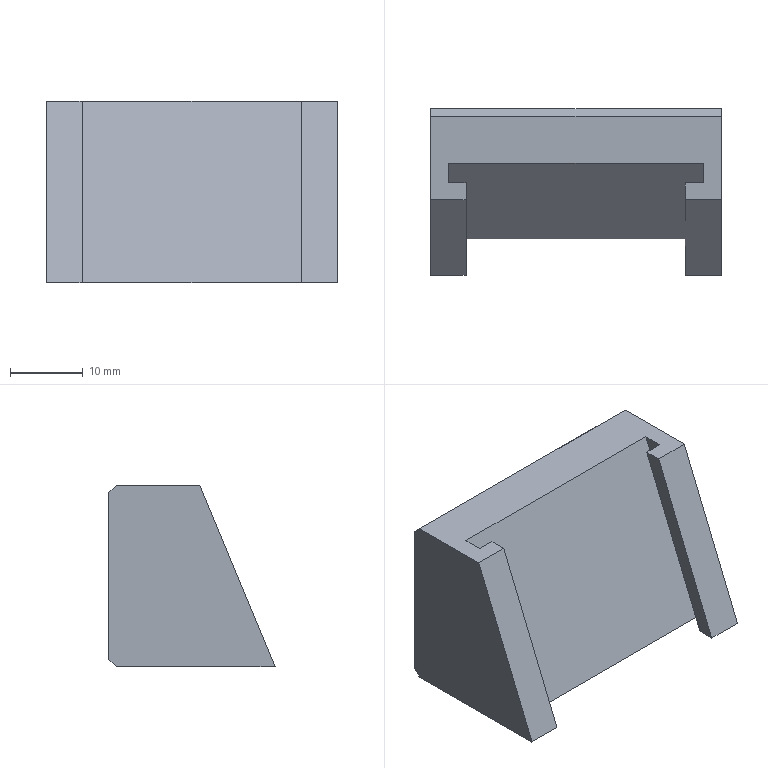Component | NX | CLAMP_SLIDER | 1 solid | 16 faces | box 40 x 22.86 x 25 mm | volume 13543 mm3 | plane 16
STEP:
#1=CARTESIAN_POINT('',(0.,0.,0.));
#2=DIRECTION('',(0.,0.,1.));
#3=DIRECTION('',(1.,0.,0.));
#4=AXIS2_PLACEMENT_3D('',#1,#2,#3);
#5=CARTESIAN_POINT('',(146.772,200.315,195.246));
#6=VERTEX_POINT('',#5);
#7=CARTESIAN_POINT('',(141.898,200.315,195.246));
#8=VERTEX_POINT('',#7);
#9=CARTESIAN_POINT('',(181.898,200.315,195.246));
#10=DIRECTION('',(-1.,0.,0.));
#11=VECTOR('',#10,1.);
#12=LINE('',#9,#11);
#13=CARTESIAN_POINT('',(181.898,200.315,195.246));
#14=DIRECTION('',(0.,-0.9239,0.3827));
#15=DIRECTION('',(0.,0.3827,0.9239));
#16=AXIS2_PLACEMENT_3D('',#13,#14,#15);
#17=PLANE('',#16);
#18=CARTESIAN_POINT('',(0.,0.));
#19=DIRECTION('',(0.,1.));
#20=VECTOR('',#19,1.);
#21=LINE('',#18,#20);
#22=(GEOMETRIC_REPRESENTATION_CONTEXT(2)PARAMETRIC_REPRESENTATION_CONTEXT()REPRESENTATION_CONTEXT('',''));
#23=DEFINITIONAL_REPRESENTATION('',(#21),#22);
#24=PCURVE('',#17,#23);
#25=CARTESIAN_POINT('',(181.898,222.171,195.246));
#26=DIRECTION('',(0.,0.,-1.));
#27=DIRECTION('',(1.,0.,0.));
#28=AXIS2_PLACEMENT_3D('',#25,#26,#27);
#29=PLANE('',#28);
#30=CARTESIAN_POINT('',(0.,21.855));
#31=DIRECTION('',(-1.,0.));
#32=VECTOR('',#31,1.);
#33=LINE('',#30,#32);
#34=(GEOMETRIC_REPRESENTATION_CONTEXT(2)PARAMETRIC_REPRESENTATION_CONTEXT()REPRESENTATION_CONTEXT('',''));
#35=DEFINITIONAL_REPRESENTATION('',(#33),#34);
#36=PCURVE('',#29,#35);
#37=SURFACE_CURVE('',#12,(#24,#36),.PCURVE_S1.);
#38=EDGE_CURVE('',#6,#8,#37,.T.);
#39=ORIENTED_EDGE('',*,*,#38,.F.);
#40=CARTESIAN_POINT('',(146.772,210.671,220.246));
#41=VERTEX_POINT('',#40);
#42=CARTESIAN_POINT('',(146.772,195.363,183.291));
#43=DIRECTION('',(0.,0.3827,0.9239));
#44=VECTOR('',#43,1.);
#45=LINE('',#42,#44);
#46=CARTESIAN_POINT('',(-12.94,35.126));
#47=DIRECTION('',(1.,0.));
#48=VECTOR('',#47,1.);
#49=LINE('',#46,#48);
#50=(GEOMETRIC_REPRESENTATION_CONTEXT(2)PARAMETRIC_REPRESENTATION_CONTEXT()REPRESENTATION_CONTEXT('',''));
#51=DEFINITIONAL_REPRESENTATION('',(#49),#50);
#52=PCURVE('',#17,#51);
#53=CARTESIAN_POINT('',(146.772,197.663,183.291));
#54=DIRECTION('',(-1.,-0.00001531,0.00000634));
#55=DIRECTION('',(0.00001531,-1.,-0.));
#56=AXIS2_PLACEMENT_3D('',#53,#54,#55);
#57=PLANE('',#56);
#58=CARTESIAN_POINT('',(2.3,0.));
#59=DIRECTION('',(-0.3827,0.9239));
#60=VECTOR('',#59,1.);
#61=LINE('',#58,#60);
#62=(GEOMETRIC_REPRESENTATION_CONTEXT(2)PARAMETRIC_REPRESENTATION_CONTEXT()REPRESENTATION_CONTEXT('',''));
#63=DEFINITIONAL_REPRESENTATION('',(#61),#62);
#64=PCURVE('',#57,#63);
#65=SURFACE_CURVE('',#45,(#52,#64),.PCURVE_S1.);
#66=EDGE_CURVE('',#6,#41,#65,.T.);
#67=ORIENTED_EDGE('',*,*,#66,.T.);
#68=CARTESIAN_POINT('',(141.898,210.671,220.246));
#69=VERTEX_POINT('',#68);
#70=CARTESIAN_POINT('',(181.898,210.671,220.246));
#71=DIRECTION('',(-1.,0.,0.));
#72=VECTOR('',#71,1.);
#73=LINE('',#70,#72);
#74=CARTESIAN_POINT('',(27.06,0.));
#75=DIRECTION('',(0.,1.));
#76=VECTOR('',#75,1.);
#77=LINE('',#74,#76);
#78=(GEOMETRIC_REPRESENTATION_CONTEXT(2)PARAMETRIC_REPRESENTATION_CONTEXT()REPRESENTATION_CONTEXT('',''));
#79=DEFINITIONAL_REPRESENTATION('',(#77),#78);
#80=PCURVE('',#17,#79);
#81=CARTESIAN_POINT('',(181.898,210.671,220.246));
#82=DIRECTION('',(0.,0.,1.));
#83=DIRECTION('',(-1.,0.,0.));
#84=AXIS2_PLACEMENT_3D('',#81,#82,#83);
#85=PLANE('',#84);
#86=CARTESIAN_POINT('',(0.,0.));
#87=DIRECTION('',(1.,0.));
#88=VECTOR('',#87,1.);
#89=LINE('',#86,#88);
#90=(GEOMETRIC_REPRESENTATION_CONTEXT(2)PARAMETRIC_REPRESENTATION_CONTEXT()REPRESENTATION_CONTEXT('',''));
#91=DEFINITIONAL_REPRESENTATION('',(#89),#90);
#92=PCURVE('',#85,#91);
#93=SURFACE_CURVE('',#73,(#80,#92),.PCURVE_S1.);
#94=EDGE_CURVE('',#41,#69,#93,.T.);
#95=ORIENTED_EDGE('',*,*,#94,.T.);
#96=CARTESIAN_POINT('',(141.898,200.315,195.246));
#97=DIRECTION('',(0.,0.3827,0.9239));
#98=VECTOR('',#97,1.);
#99=LINE('',#96,#98);
#100=CARTESIAN_POINT('',(0.,40.));
#101=DIRECTION('',(1.,0.));
#102=VECTOR('',#101,1.);
#103=LINE('',#100,#102);
#104=(GEOMETRIC_REPRESENTATION_CONTEXT(2)PARAMETRIC_REPRESENTATION_CONTEXT()REPRESENTATION_CONTEXT('',''));
#105=DEFINITIONAL_REPRESENTATION('',(#103),#104);
#106=PCURVE('',#17,#105);
#107=CARTESIAN_POINT('',(141.898,223.171,220.246));
#108=DIRECTION('',(-1.,0.,0.));
#109=DIRECTION('',(0.,0.,-1.));
#110=AXIS2_PLACEMENT_3D('',#107,#108,#109);
#111=PLANE('',#110);
#112=CARTESIAN_POINT('',(25.,22.855));
#113=DIRECTION('',(-0.9239,-0.3827));
#114=VECTOR('',#113,1.);
#115=LINE('',#112,#114);
#116=(GEOMETRIC_REPRESENTATION_CONTEXT(2)PARAMETRIC_REPRESENTATION_CONTEXT()REPRESENTATION_CONTEXT('',''));
#117=DEFINITIONAL_REPRESENTATION('',(#115),#116);
#118=PCURVE('',#111,#117);
#119=SURFACE_CURVE('',#99,(#106,#118),.PCURVE_S1.);
#120=EDGE_CURVE('',#8,#69,#119,.T.);
#121=ORIENTED_EDGE('',*,*,#120,.F.);
#122=EDGE_LOOP('',(#39,#67,#95,#121));
#123=FACE_BOUND('',#122,.T.);
#124=ADVANCED_FACE('',(#123),#17,.T.);
#125=CARTESIAN_POINT('',(141.898,223.171,219.246));
#126=VERTEX_POINT('',#125);
#127=CARTESIAN_POINT('',(141.898,223.171,196.246));
#128=VERTEX_POINT('',#127);
#129=CARTESIAN_POINT('',(141.898,223.171,219.246));
#130=DIRECTION('',(0.,0.,-1.));
#131=VECTOR('',#130,1.);
#132=LINE('',#129,#131);
#133=CARTESIAN_POINT('',(181.898,223.171,219.246));
#134=DIRECTION('',(0.,1.,0.));
#135=DIRECTION('',(0.,0.,-1.));
#136=AXIS2_PLACEMENT_3D('',#133,#134,#135);
#137=PLANE('',#136);
#138=CARTESIAN_POINT('',(0.,40.));
#139=DIRECTION('',(1.,0.));
#140=VECTOR('',#139,1.);
#141=LINE('',#138,#140);
#142=(GEOMETRIC_REPRESENTATION_CONTEXT(2)PARAMETRIC_REPRESENTATION_CONTEXT()REPRESENTATION_CONTEXT('',''));
#143=DEFINITIONAL_REPRESENTATION('',(#141),#142);
#144=PCURVE('',#137,#143);
#145=CARTESIAN_POINT('',(1.,0.));
#146=DIRECTION('',(1.,-0.));
#147=VECTOR('',#146,1.);
#148=LINE('',#145,#147);
#149=(GEOMETRIC_REPRESENTATION_CONTEXT(2)PARAMETRIC_REPRESENTATION_CONTEXT()REPRESENTATION_CONTEXT('',''));
#150=DEFINITIONAL_REPRESENTATION('',(#148),#149);
#151=PCURVE('',#111,#150);
#152=SURFACE_CURVE('',#132,(#144,#151),.PCURVE_S1.);
#153=EDGE_CURVE('',#126,#128,#152,.T.);
#154=ORIENTED_EDGE('',*,*,#153,.F.);
#155=CARTESIAN_POINT('',(181.898,223.171,219.246));
#156=VERTEX_POINT('',#155);
#157=CARTESIAN_POINT('',(181.898,223.171,219.246));
#158=DIRECTION('',(-1.,0.,0.));
#159=VECTOR('',#158,1.);
#160=LINE('',#157,#159);
#161=CARTESIAN_POINT('',(0.,0.));
#162=DIRECTION('',(0.,1.));
#163=VECTOR('',#162,1.);
#164=LINE('',#161,#163);
#165=(GEOMETRIC_REPRESENTATION_CONTEXT(2)PARAMETRIC_REPRESENTATION_CONTEXT()REPRESENTATION_CONTEXT('',''));
#166=DEFINITIONAL_REPRESENTATION('',(#164),#165);
#167=PCURVE('',#137,#166);
#168=CARTESIAN_POINT('',(181.898,222.171,220.246));
#169=DIRECTION('',(0.,0.7071,0.7071));
#170=DIRECTION('',(0.,0.7071,-0.7071));
#171=AXIS2_PLACEMENT_3D('',#168,#169,#170);
#172=PLANE('',#171);
#173=CARTESIAN_POINT('',(1.414,0.));
#174=DIRECTION('',(0.,1.));
#175=VECTOR('',#174,1.);
#176=LINE('',#173,#175);
#177=(GEOMETRIC_REPRESENTATION_CONTEXT(2)PARAMETRIC_REPRESENTATION_CONTEXT()REPRESENTATION_CONTEXT('',''));
#178=DEFINITIONAL_REPRESENTATION('',(#176),#177);
#179=PCURVE('',#172,#178);
#180=SURFACE_CURVE('',#160,(#167,#179),.PCURVE_S1.);
#181=EDGE_CURVE('',#156,#126,#180,.T.);
#182=ORIENTED_EDGE('',*,*,#181,.F.);
#183=CARTESIAN_POINT('',(181.898,223.171,196.246));
#184=VERTEX_POINT('',#183);
#185=CARTESIAN_POINT('',(181.898,223.171,219.246));
#186=DIRECTION('',(0.,0.,-1.));
#187=VECTOR('',#186,1.);
#188=LINE('',#185,#187);
#189=CARTESIAN_POINT('',(0.,0.));
#190=DIRECTION('',(1.,0.));
#191=VECTOR('',#190,1.);
#192=LINE('',#189,#191);
#193=(GEOMETRIC_REPRESENTATION_CONTEXT(2)PARAMETRIC_REPRESENTATION_CONTEXT()REPRESENTATION_CONTEXT('',''));
#194=DEFINITIONAL_REPRESENTATION('',(#192),#193);
#195=PCURVE('',#137,#194);
#196=CARTESIAN_POINT('',(181.898,223.171,220.246));
#197=DIRECTION('',(-1.,0.,0.));
#198=DIRECTION('',(0.,0.,-1.));
#199=AXIS2_PLACEMENT_3D('',#196,#197,#198);
#200=PLANE('',#199);
#201=CARTESIAN_POINT('',(1.,0.));
#202=DIRECTION('',(1.,-0.));
#203=VECTOR('',#202,1.);
#204=LINE('',#201,#203);
#205=(GEOMETRIC_REPRESENTATION_CONTEXT(2)PARAMETRIC_REPRESENTATION_CONTEXT()REPRESENTATION_CONTEXT('',''));
#206=DEFINITIONAL_REPRESENTATION('',(#204),#205);
#207=PCURVE('',#200,#206);
#208=SURFACE_CURVE('',#188,(#195,#207),.PCURVE_S1.);
#209=EDGE_CURVE('',#156,#184,#208,.T.);
#210=ORIENTED_EDGE('',*,*,#209,.T.);
#211=CARTESIAN_POINT('',(181.898,223.171,196.246));
#212=DIRECTION('',(-1.,0.,0.));
#213=VECTOR('',#212,1.);
#214=LINE('',#211,#213);
#215=CARTESIAN_POINT('',(23.,0.));
#216=DIRECTION('',(0.,1.));
#217=VECTOR('',#216,1.);
#218=LINE('',#215,#217);
#219=(GEOMETRIC_REPRESENTATION_CONTEXT(2)PARAMETRIC_REPRESENTATION_CONTEXT()REPRESENTATION_CONTEXT('',''));
#220=DEFINITIONAL_REPRESENTATION('',(#218),#219);
#221=PCURVE('',#137,#220);
#222=CARTESIAN_POINT('',(181.898,223.171,196.246));
#223=DIRECTION('',(0.,0.7071,-0.7071));
#224=DIRECTION('',(0.,-0.7071,-0.7071));
#225=AXIS2_PLACEMENT_3D('',#222,#223,#224);
#226=PLANE('',#225);
#227=CARTESIAN_POINT('',(0.,0.));
#228=DIRECTION('',(0.,1.));
#229=VECTOR('',#228,1.);
#230=LINE('',#227,#229);
#231=(GEOMETRIC_REPRESENTATION_CONTEXT(2)PARAMETRIC_REPRESENTATION_CONTEXT()REPRESENTATION_CONTEXT('',''));
#232=DEFINITIONAL_REPRESENTATION('',(#230),#231);
#233=PCURVE('',#226,#232);
#234=SURFACE_CURVE('',#214,(#221,#233),.PCURVE_S1.);
#235=EDGE_CURVE('',#184,#128,#234,.T.);
#236=ORIENTED_EDGE('',*,*,#235,.T.);
#237=EDGE_LOOP('',(#154,#182,#210,#236));
#238=FACE_BOUND('',#237,.T.);
#239=ADVANCED_FACE('',(#238),#137,.T.);
#240=CARTESIAN_POINT('',(141.898,222.171,195.246));
#241=VERTEX_POINT('',#240);
#242=CARTESIAN_POINT('',(141.898,223.171,196.246));
#243=DIRECTION('',(0.,-0.7071,-0.7071));
#244=VECTOR('',#243,1.);
#245=LINE('',#242,#244);
#246=CARTESIAN_POINT('',(0.,40.));
#247=DIRECTION('',(1.,0.));
#248=VECTOR('',#247,1.);
#249=LINE('',#246,#248);
#250=(GEOMETRIC_REPRESENTATION_CONTEXT(2)PARAMETRIC_REPRESENTATION_CONTEXT()REPRESENTATION_CONTEXT('',''));
#251=DEFINITIONAL_REPRESENTATION('',(#249),#250);
#252=PCURVE('',#226,#251);
#253=CARTESIAN_POINT('',(24.,0.));
#254=DIRECTION('',(0.7071,0.7071));
#255=VECTOR('',#254,1.);
#256=LINE('',#253,#255);
#257=(GEOMETRIC_REPRESENTATION_CONTEXT(2)PARAMETRIC_REPRESENTATION_CONTEXT()REPRESENTATION_CONTEXT('',''));
#258=DEFINITIONAL_REPRESENTATION('',(#256),#257);
#259=PCURVE('',#111,#258);
#260=SURFACE_CURVE('',#245,(#252,#259),.PCURVE_S1.);
#261=EDGE_CURVE('',#128,#241,#260,.T.);
#262=ORIENTED_EDGE('',*,*,#261,.F.);
#263=ORIENTED_EDGE('',*,*,#235,.F.);
#264=CARTESIAN_POINT('',(181.898,222.171,195.246));
#265=VERTEX_POINT('',#264);
#266=CARTESIAN_POINT('',(181.898,223.171,196.246));
#267=DIRECTION('',(0.,-0.7071,-0.7071));
#268=VECTOR('',#267,1.);
#269=LINE('',#266,#268);
#270=CARTESIAN_POINT('',(0.,0.));
#271=DIRECTION('',(1.,0.));
#272=VECTOR('',#271,1.);
#273=LINE('',#270,#272);
#274=(GEOMETRIC_REPRESENTATION_CONTEXT(2)PARAMETRIC_REPRESENTATION_CONTEXT()REPRESENTATION_CONTEXT('',''));
#275=DEFINITIONAL_REPRESENTATION('',(#273),#274);
#276=PCURVE('',#226,#275);
#277=CARTESIAN_POINT('',(24.,0.));
#278=DIRECTION('',(0.7071,0.7071));
#279=VECTOR('',#278,1.);
#280=LINE('',#277,#279);
#281=(GEOMETRIC_REPRESENTATION_CONTEXT(2)PARAMETRIC_REPRESENTATION_CONTEXT()REPRESENTATION_CONTEXT('',''));
#282=DEFINITIONAL_REPRESENTATION('',(#280),#281);
#283=PCURVE('',#200,#282);
#284=SURFACE_CURVE('',#269,(#276,#283),.PCURVE_S1.);
#285=EDGE_CURVE('',#184,#265,#284,.T.);
#286=ORIENTED_EDGE('',*,*,#285,.T.);
#287=CARTESIAN_POINT('',(181.898,222.171,195.246));
#288=DIRECTION('',(-1.,0.,0.));
#289=VECTOR('',#288,1.);
#290=LINE('',#287,#289);
#291=CARTESIAN_POINT('',(1.414,0.));
#292=DIRECTION('',(0.,1.));
#293=VECTOR('',#292,1.);
#294=LINE('',#291,#293);
#295=(GEOMETRIC_REPRESENTATION_CONTEXT(2)PARAMETRIC_REPRESENTATION_CONTEXT()REPRESENTATION_CONTEXT('',''));
#296=DEFINITIONAL_REPRESENTATION('',(#294),#295);
#297=PCURVE('',#226,#296);
#298=CARTESIAN_POINT('',(0.,0.));
#299=DIRECTION('',(-1.,0.));
#300=VECTOR('',#299,1.);
#301=LINE('',#298,#300);
#302=(GEOMETRIC_REPRESENTATION_CONTEXT(2)PARAMETRIC_REPRESENTATION_CONTEXT()REPRESENTATION_CONTEXT('',''));
#303=DEFINITIONAL_REPRESENTATION('',(#301),#302);
#304=PCURVE('',#29,#303);
#305=SURFACE_CURVE('',#290,(#297,#304),.PCURVE_S1.);
#306=EDGE_CURVE('',#265,#241,#305,.T.);
#307=ORIENTED_EDGE('',*,*,#306,.T.);
#308=EDGE_LOOP('',(#262,#263,#286,#307));
#309=FACE_BOUND('',#308,.T.);
#310=ADVANCED_FACE('',(#309),#226,.T.);
#311=CARTESIAN_POINT('',(146.772,202.615,195.246));
#312=VERTEX_POINT('',#311);
#313=CARTESIAN_POINT('',(146.771,222.17,195.246));
#314=DIRECTION('',(-0.00001531,1.,0.));
#315=VECTOR('',#314,1.);
#316=LINE('',#313,#315);
#317=CARTESIAN_POINT('',(-35.126,0.0005376));
#318=DIRECTION('',(-0.00001531,-1.));
#319=VECTOR('',#318,1.);
#320=LINE('',#317,#319);
#321=(GEOMETRIC_REPRESENTATION_CONTEXT(2)PARAMETRIC_REPRESENTATION_CONTEXT()REPRESENTATION_CONTEXT('',''));
#322=DEFINITIONAL_REPRESENTATION('',(#320),#321);
#323=PCURVE('',#29,#322);
#324=CARTESIAN_POINT('',(-24.507,11.955));
#325=DIRECTION('',(-1.,-0.));
#326=VECTOR('',#325,1.);
#327=LINE('',#324,#326);
#328=(GEOMETRIC_REPRESENTATION_CONTEXT(2)PARAMETRIC_REPRESENTATION_CONTEXT()REPRESENTATION_CONTEXT('',''));
#329=DEFINITIONAL_REPRESENTATION('',(#327),#328);
#330=PCURVE('',#57,#329);
#331=SURFACE_CURVE('',#316,(#323,#330),.PCURVE_S1.);
#332=EDGE_CURVE('',#6,#312,#331,.T.);
#333=ORIENTED_EDGE('',*,*,#332,.F.);
#334=ORIENTED_EDGE('',*,*,#38,.T.);
#335=CARTESIAN_POINT('',(141.898,222.171,195.246));
#336=DIRECTION('',(0.,-1.,0.));
#337=VECTOR('',#336,1.);
#338=LINE('',#335,#337);
#339=CARTESIAN_POINT('',(-40.,0.));
#340=DIRECTION('',(0.,1.));
#341=VECTOR('',#340,1.);
#342=LINE('',#339,#341);
#343=(GEOMETRIC_REPRESENTATION_CONTEXT(2)PARAMETRIC_REPRESENTATION_CONTEXT()REPRESENTATION_CONTEXT('',''));
#344=DEFINITIONAL_REPRESENTATION('',(#342),#343);
#345=PCURVE('',#29,#344);
#346=CARTESIAN_POINT('',(25.,1.));
#347=DIRECTION('',(0.,1.));
#348=VECTOR('',#347,1.);
#349=LINE('',#346,#348);
#350=(GEOMETRIC_REPRESENTATION_CONTEXT(2)PARAMETRIC_REPRESENTATION_CONTEXT()REPRESENTATION_CONTEXT('',''));
#351=DEFINITIONAL_REPRESENTATION('',(#349),#350);
#352=PCURVE('',#111,#351);
#353=SURFACE_CURVE('',#338,(#345,#352),.PCURVE_S1.);
#354=EDGE_CURVE('',#241,#8,#353,.T.);
#355=ORIENTED_EDGE('',*,*,#354,.F.);
#356=ORIENTED_EDGE('',*,*,#306,.F.);
#357=CARTESIAN_POINT('',(181.898,200.315,195.246));
#358=VERTEX_POINT('',#357);
#359=CARTESIAN_POINT('',(181.898,222.171,195.246));
#360=DIRECTION('',(0.,-1.,0.));
#361=VECTOR('',#360,1.);
#362=LINE('',#359,#361);
#363=CARTESIAN_POINT('',(0.,0.));
#364=DIRECTION('',(0.,1.));
#365=VECTOR('',#364,1.);
#366=LINE('',#363,#365);
#367=(GEOMETRIC_REPRESENTATION_CONTEXT(2)PARAMETRIC_REPRESENTATION_CONTEXT()REPRESENTATION_CONTEXT('',''));
#368=DEFINITIONAL_REPRESENTATION('',(#366),#367);
#369=PCURVE('',#29,#368);
#370=CARTESIAN_POINT('',(25.,1.));
#371=DIRECTION('',(0.,1.));
#372=VECTOR('',#371,1.);
#373=LINE('',#370,#372);
#374=(GEOMETRIC_REPRESENTATION_CONTEXT(2)PARAMETRIC_REPRESENTATION_CONTEXT()REPRESENTATION_CONTEXT('',''));
#375=DEFINITIONAL_REPRESENTATION('',(#373),#374);
#376=PCURVE('',#200,#375);
#377=SURFACE_CURVE('',#362,(#369,#376),.PCURVE_S1.);
#378=EDGE_CURVE('',#265,#358,#377,.T.);
#379=ORIENTED_EDGE('',*,*,#378,.T.);
#380=CARTESIAN_POINT('',(176.898,200.315,195.246));
#381=VERTEX_POINT('',#380);
#382=CARTESIAN_POINT('',(181.898,200.315,195.246));
#383=DIRECTION('',(-1.,0.,0.));
#384=VECTOR('',#383,1.);
#385=LINE('',#382,#384);
#386=CARTESIAN_POINT('',(0.,21.855));
#387=DIRECTION('',(-1.,0.));
#388=VECTOR('',#387,1.);
#389=LINE('',#386,#388);
#390=(GEOMETRIC_REPRESENTATION_CONTEXT(2)PARAMETRIC_REPRESENTATION_CONTEXT()REPRESENTATION_CONTEXT('',''));
#391=DEFINITIONAL_REPRESENTATION('',(#389),#390);
#392=PCURVE('',#29,#391);
#393=CARTESIAN_POINT('',(181.898,200.315,195.246));
#394=DIRECTION('',(0.,-0.9239,0.3827));
#395=DIRECTION('',(0.,0.3827,0.9239));
#396=AXIS2_PLACEMENT_3D('',#393,#394,#395);
#397=PLANE('',#396);
#398=CARTESIAN_POINT('',(0.,0.));
#399=DIRECTION('',(0.,1.));
#400=VECTOR('',#399,1.);
#401=LINE('',#398,#400);
#402=(GEOMETRIC_REPRESENTATION_CONTEXT(2)PARAMETRIC_REPRESENTATION_CONTEXT()REPRESENTATION_CONTEXT('',''));
#403=DEFINITIONAL_REPRESENTATION('',(#401),#402);
#404=PCURVE('',#397,#403);
#405=SURFACE_CURVE('',#385,(#392,#404),.PCURVE_S1.);
#406=EDGE_CURVE('',#358,#381,#405,.T.);
#407=ORIENTED_EDGE('',*,*,#406,.T.);
#408=CARTESIAN_POINT('',(176.898,202.615,195.246));
#409=VERTEX_POINT('',#408);
#410=CARTESIAN_POINT('',(176.898,222.171,195.246));
#411=DIRECTION('',(0.,-1.,0.));
#412=VECTOR('',#411,1.);
#413=LINE('',#410,#412);
#414=CARTESIAN_POINT('',(-5.,0.));
#415=DIRECTION('',(0.,1.));
#416=VECTOR('',#415,1.);
#417=LINE('',#414,#416);
#418=(GEOMETRIC_REPRESENTATION_CONTEXT(2)PARAMETRIC_REPRESENTATION_CONTEXT()REPRESENTATION_CONTEXT('',''));
#419=DEFINITIONAL_REPRESENTATION('',(#417),#418);
#420=PCURVE('',#29,#419);
#421=CARTESIAN_POINT('',(176.898,195.363,183.291));
#422=DIRECTION('',(1.,0.,0.));
#423=DIRECTION('',(0.,0.,1.));
#424=AXIS2_PLACEMENT_3D('',#421,#422,#423);
#425=PLANE('',#424);
#426=CARTESIAN_POINT('',(11.955,-26.807));
#427=DIRECTION('',(0.,1.));
#428=VECTOR('',#427,1.);
#429=LINE('',#426,#428);
#430=(GEOMETRIC_REPRESENTATION_CONTEXT(2)PARAMETRIC_REPRESENTATION_CONTEXT()REPRESENTATION_CONTEXT('',''));
#431=DEFINITIONAL_REPRESENTATION('',(#429),#430);
#432=PCURVE('',#425,#431);
#433=SURFACE_CURVE('',#413,(#420,#432),.PCURVE_S1.);
#434=EDGE_CURVE('',#409,#381,#433,.T.);
#435=ORIENTED_EDGE('',*,*,#434,.F.);
#436=CARTESIAN_POINT('',(179.398,202.615,195.246));
#437=VERTEX_POINT('',#436);
#438=CARTESIAN_POINT('',(181.898,202.615,195.246));
#439=DIRECTION('',(-1.,0.,0.));
#440=VECTOR('',#439,1.);
#441=LINE('',#438,#440);
#442=CARTESIAN_POINT('',(0.,19.555));
#443=DIRECTION('',(-1.,0.));
#444=VECTOR('',#443,1.);
#445=LINE('',#442,#444);
#446=(GEOMETRIC_REPRESENTATION_CONTEXT(2)PARAMETRIC_REPRESENTATION_CONTEXT()REPRESENTATION_CONTEXT('',''));
#447=DEFINITIONAL_REPRESENTATION('',(#445),#446);
#448=PCURVE('',#29,#447);
#449=CARTESIAN_POINT('',(176.898,197.663,183.291));
#450=DIRECTION('',(0.,-0.9239,0.3827));
#451=DIRECTION('',(0.,0.3827,0.9239));
#452=AXIS2_PLACEMENT_3D('',#449,#450,#451);
#453=PLANE('',#452);
#454=CARTESIAN_POINT('',(12.94,-5.));
#455=DIRECTION('',(0.,1.));
#456=VECTOR('',#455,1.);
#457=LINE('',#454,#456);
#458=(GEOMETRIC_REPRESENTATION_CONTEXT(2)PARAMETRIC_REPRESENTATION_CONTEXT()REPRESENTATION_CONTEXT('',''));
#459=DEFINITIONAL_REPRESENTATION('',(#457),#458);
#460=PCURVE('',#453,#459);
#461=SURFACE_CURVE('',#441,(#448,#460),.PCURVE_S1.);
#462=EDGE_CURVE('',#437,#409,#461,.T.);
#463=ORIENTED_EDGE('',*,*,#462,.F.);
#464=CARTESIAN_POINT('',(179.398,205.315,195.246));
#465=VERTEX_POINT('',#464);
#466=CARTESIAN_POINT('',(179.398,222.171,195.246));
#467=DIRECTION('',(-0.,-1.,0.));
#468=VECTOR('',#467,1.);
#469=LINE('',#466,#468);
#470=CARTESIAN_POINT('',(-2.5,0.));
#471=DIRECTION('',(-0.,1.));
#472=VECTOR('',#471,1.);
#473=LINE('',#470,#472);
#474=(GEOMETRIC_REPRESENTATION_CONTEXT(2)PARAMETRIC_REPRESENTATION_CONTEXT()REPRESENTATION_CONTEXT('',''));
#475=DEFINITIONAL_REPRESENTATION('',(#473),#474);
#476=PCURVE('',#29,#475);
#477=CARTESIAN_POINT('',(179.398,197.663,183.291));
#478=DIRECTION('',(1.,-0.,0.));
#479=DIRECTION('',(0.,1.,0.));
#480=AXIS2_PLACEMENT_3D('',#477,#478,#479);
#481=PLANE('',#480);
#482=CARTESIAN_POINT('',(24.507,11.955));
#483=DIRECTION('',(-1.,0.));
#484=VECTOR('',#483,1.);
#485=LINE('',#482,#484);
#486=(GEOMETRIC_REPRESENTATION_CONTEXT(2)PARAMETRIC_REPRESENTATION_CONTEXT()REPRESENTATION_CONTEXT('',''));
#487=DEFINITIONAL_REPRESENTATION('',(#485),#486);
#488=PCURVE('',#481,#487);
#489=SURFACE_CURVE('',#469,(#476,#488),.PCURVE_S1.);
#490=EDGE_CURVE('',#465,#437,#489,.T.);
#491=ORIENTED_EDGE('',*,*,#490,.F.);
#492=CARTESIAN_POINT('',(144.398,205.315,195.246));
#493=VERTEX_POINT('',#492);
#494=CARTESIAN_POINT('',(181.898,205.315,195.246));
#495=DIRECTION('',(1.,-0.,0.));
#496=VECTOR('',#495,1.);
#497=LINE('',#494,#496);
#498=CARTESIAN_POINT('',(0.,16.855));
#499=DIRECTION('',(1.,0.));
#500=VECTOR('',#499,1.);
#501=LINE('',#498,#500);
#502=(GEOMETRIC_REPRESENTATION_CONTEXT(2)PARAMETRIC_REPRESENTATION_CONTEXT()REPRESENTATION_CONTEXT('',''));
#503=DEFINITIONAL_REPRESENTATION('',(#501),#502);
#504=PCURVE('',#29,#503);
#505=CARTESIAN_POINT('',(161.898,200.363,183.291));
#506=DIRECTION('',(0.,0.9239,-0.3827));
#507=DIRECTION('',(-0.,-0.3827,-0.9239));
#508=AXIS2_PLACEMENT_3D('',#505,#506,#507);
#509=PLANE('',#508);
#510=CARTESIAN_POINT('',(-12.94,-20.));
#511=DIRECTION('',(0.,-1.));
#512=VECTOR('',#511,1.);
#513=LINE('',#510,#512);
#514=(GEOMETRIC_REPRESENTATION_CONTEXT(2)PARAMETRIC_REPRESENTATION_CONTEXT()REPRESENTATION_CONTEXT('',''));
#515=DEFINITIONAL_REPRESENTATION('',(#513),#514);
#516=PCURVE('',#509,#515);
#517=SURFACE_CURVE('',#497,(#504,#516),.PCURVE_S1.);
#518=EDGE_CURVE('',#493,#465,#517,.T.);
#519=ORIENTED_EDGE('',*,*,#518,.F.);
#520=CARTESIAN_POINT('',(144.398,202.615,195.246));
#521=VERTEX_POINT('',#520);
#522=CARTESIAN_POINT('',(144.398,222.171,195.246));
#523=DIRECTION('',(0.,1.,0.));
#524=VECTOR('',#523,1.);
#525=LINE('',#522,#524);
#526=CARTESIAN_POINT('',(-37.5,0.));
#527=DIRECTION('',(0.,-1.));
#528=VECTOR('',#527,1.);
#529=LINE('',#526,#528);
#530=(GEOMETRIC_REPRESENTATION_CONTEXT(2)PARAMETRIC_REPRESENTATION_CONTEXT()REPRESENTATION_CONTEXT('',''));
#531=DEFINITIONAL_REPRESENTATION('',(#529),#530);
#532=PCURVE('',#29,#531);
#533=CARTESIAN_POINT('',(144.398,200.363,183.291));
#534=DIRECTION('',(-1.,0.,-0.));
#535=DIRECTION('',(-0.,-1.,0.));
#536=AXIS2_PLACEMENT_3D('',#533,#534,#535);
#537=PLANE('',#536);
#538=CARTESIAN_POINT('',(-21.807,11.955));
#539=DIRECTION('',(-1.,0.));
#540=VECTOR('',#539,1.);
#541=LINE('',#538,#540);
#542=(GEOMETRIC_REPRESENTATION_CONTEXT(2)PARAMETRIC_REPRESENTATION_CONTEXT()REPRESENTATION_CONTEXT('',''));
#543=DEFINITIONAL_REPRESENTATION('',(#541),#542);
#544=PCURVE('',#537,#543);
#545=SURFACE_CURVE('',#525,(#532,#544),.PCURVE_S1.);
#546=EDGE_CURVE('',#521,#493,#545,.T.);
#547=ORIENTED_EDGE('',*,*,#546,.F.);
#548=CARTESIAN_POINT('',(181.898,202.615,195.246));
#549=DIRECTION('',(-1.,0.,0.));
#550=VECTOR('',#549,1.);
#551=LINE('',#548,#550);
#552=CARTESIAN_POINT('',(0.,19.555));
#553=DIRECTION('',(-1.,0.));
#554=VECTOR('',#553,1.);
#555=LINE('',#552,#554);
#556=(GEOMETRIC_REPRESENTATION_CONTEXT(2)PARAMETRIC_REPRESENTATION_CONTEXT()REPRESENTATION_CONTEXT('',''));
#557=DEFINITIONAL_REPRESENTATION('',(#555),#556);
#558=PCURVE('',#29,#557);
#559=CARTESIAN_POINT('',(144.398,197.663,183.291));
#560=DIRECTION('',(0.,-0.9239,0.3827));
#561=DIRECTION('',(0.,0.3827,0.9239));
#562=AXIS2_PLACEMENT_3D('',#559,#560,#561);
#563=PLANE('',#562);
#564=CARTESIAN_POINT('',(12.94,-37.5));
#565=DIRECTION('',(0.,1.));
#566=VECTOR('',#565,1.);
#567=LINE('',#564,#566);
#568=(GEOMETRIC_REPRESENTATION_CONTEXT(2)PARAMETRIC_REPRESENTATION_CONTEXT()REPRESENTATION_CONTEXT('',''));
#569=DEFINITIONAL_REPRESENTATION('',(#567),#568);
#570=PCURVE('',#563,#569);
#571=SURFACE_CURVE('',#551,(#558,#570),.PCURVE_S1.);
#572=EDGE_CURVE('',#312,#521,#571,.T.);
#573=ORIENTED_EDGE('',*,*,#572,.F.);
#574=EDGE_LOOP('',(#333,#334,#355,#356,#379,#407,#435,#463,#491,#519,#547,#573));
#575=FACE_BOUND('',#574,.T.);
#576=ADVANCED_FACE('',(#575),#29,.T.);
#577=CARTESIAN_POINT('',(176.898,210.671,220.246));
#578=VERTEX_POINT('',#577);
#579=CARTESIAN_POINT('',(176.898,195.363,183.291));
#580=DIRECTION('',(0.,0.3827,0.9239));
#581=VECTOR('',#580,1.);
#582=LINE('',#579,#581);
#583=CARTESIAN_POINT('',(-12.94,5.));
#584=DIRECTION('',(1.,0.));
#585=VECTOR('',#584,1.);
#586=LINE('',#583,#585);
#587=(GEOMETRIC_REPRESENTATION_CONTEXT(2)PARAMETRIC_REPRESENTATION_CONTEXT()REPRESENTATION_CONTEXT('',''));
#588=DEFINITIONAL_REPRESENTATION('',(#586),#587);
#589=PCURVE('',#397,#588);
#590=CARTESIAN_POINT('',(0.,0.));
#591=DIRECTION('',(0.9239,-0.3827));
#592=VECTOR('',#591,1.);
#593=LINE('',#590,#592);
#594=(GEOMETRIC_REPRESENTATION_CONTEXT(2)PARAMETRIC_REPRESENTATION_CONTEXT()REPRESENTATION_CONTEXT('',''));
#595=DEFINITIONAL_REPRESENTATION('',(#593),#594);
#596=PCURVE('',#425,#595);
#597=SURFACE_CURVE('',#582,(#589,#596),.PCURVE_S1.);
#598=EDGE_CURVE('',#381,#578,#597,.T.);
#599=ORIENTED_EDGE('',*,*,#598,.F.);
#600=ORIENTED_EDGE('',*,*,#406,.F.);
#601=CARTESIAN_POINT('',(181.898,210.671,220.246));
#602=VERTEX_POINT('',#601);
#603=CARTESIAN_POINT('',(181.898,200.315,195.246));
#604=DIRECTION('',(0.,0.3827,0.9239));
#605=VECTOR('',#604,1.);
#606=LINE('',#603,#605);
#607=CARTESIAN_POINT('',(0.,0.));
#608=DIRECTION('',(1.,0.));
#609=VECTOR('',#608,1.);
#610=LINE('',#607,#609);
#611=(GEOMETRIC_REPRESENTATION_CONTEXT(2)PARAMETRIC_REPRESENTATION_CONTEXT()REPRESENTATION_CONTEXT('',''));
#612=DEFINITIONAL_REPRESENTATION('',(#610),#611);
#613=PCURVE('',#397,#612);
#614=CARTESIAN_POINT('',(25.,22.855));
#615=DIRECTION('',(-0.9239,-0.3827));
#616=VECTOR('',#615,1.);
#617=LINE('',#614,#616);
#618=(GEOMETRIC_REPRESENTATION_CONTEXT(2)PARAMETRIC_REPRESENTATION_CONTEXT()REPRESENTATION_CONTEXT('',''));
#619=DEFINITIONAL_REPRESENTATION('',(#617),#618);
#620=PCURVE('',#200,#619);
#621=SURFACE_CURVE('',#606,(#613,#620),.PCURVE_S1.);
#622=EDGE_CURVE('',#358,#602,#621,.T.);
#623=ORIENTED_EDGE('',*,*,#622,.T.);
#624=CARTESIAN_POINT('',(181.898,210.671,220.246));
#625=DIRECTION('',(-1.,0.,0.));
#626=VECTOR('',#625,1.);
#627=LINE('',#624,#626);
#628=CARTESIAN_POINT('',(27.06,0.));
#629=DIRECTION('',(0.,1.));
#630=VECTOR('',#629,1.);
#631=LINE('',#628,#630);
#632=(GEOMETRIC_REPRESENTATION_CONTEXT(2)PARAMETRIC_REPRESENTATION_CONTEXT()REPRESENTATION_CONTEXT('',''));
#633=DEFINITIONAL_REPRESENTATION('',(#631),#632);
#634=PCURVE('',#397,#633);
#635=CARTESIAN_POINT('',(0.,0.));
#636=DIRECTION('',(1.,0.));
#637=VECTOR('',#636,1.);
#638=LINE('',#635,#637);
#639=(GEOMETRIC_REPRESENTATION_CONTEXT(2)PARAMETRIC_REPRESENTATION_CONTEXT()REPRESENTATION_CONTEXT('',''));
#640=DEFINITIONAL_REPRESENTATION('',(#638),#639);
#641=PCURVE('',#85,#640);
#642=SURFACE_CURVE('',#627,(#634,#641),.PCURVE_S1.);
#643=EDGE_CURVE('',#602,#578,#642,.T.);
#644=ORIENTED_EDGE('',*,*,#643,.T.);
#645=EDGE_LOOP('',(#599,#600,#623,#644));
#646=FACE_BOUND('',#645,.T.);
#647=ADVANCED_FACE('',(#646),#397,.T.);
#648=CARTESIAN_POINT('',(176.898,212.971,220.246));
#649=VERTEX_POINT('',#648);
#650=CARTESIAN_POINT('',(176.898,210.671,220.246));
#651=DIRECTION('',(0.,1.,0.));
#652=VECTOR('',#651,1.);
#653=LINE('',#650,#652);
#654=CARTESIAN_POINT('',(5.,0.));
#655=DIRECTION('',(0.,-1.));
#656=VECTOR('',#655,1.);
#657=LINE('',#654,#656);
#658=(GEOMETRIC_REPRESENTATION_CONTEXT(2)PARAMETRIC_REPRESENTATION_CONTEXT()REPRESENTATION_CONTEXT('',''));
#659=DEFINITIONAL_REPRESENTATION('',(#657),#658);
#660=PCURVE('',#85,#659);
#661=CARTESIAN_POINT('',(36.955,-15.307));
#662=DIRECTION('',(0.,-1.));
#663=VECTOR('',#662,1.);
#664=LINE('',#661,#663);
#665=(GEOMETRIC_REPRESENTATION_CONTEXT(2)PARAMETRIC_REPRESENTATION_CONTEXT()REPRESENTATION_CONTEXT('',''));
#666=DEFINITIONAL_REPRESENTATION('',(#664),#665);
#667=PCURVE('',#425,#666);
#668=SURFACE_CURVE('',#653,(#660,#667),.PCURVE_S1.);
#669=EDGE_CURVE('',#578,#649,#668,.T.);
#670=ORIENTED_EDGE('',*,*,#669,.F.);
#671=ORIENTED_EDGE('',*,*,#643,.F.);
#672=CARTESIAN_POINT('',(181.898,222.171,220.246));
#673=VERTEX_POINT('',#672);
#674=CARTESIAN_POINT('',(181.898,210.671,220.246));
#675=DIRECTION('',(0.,1.,0.));
#676=VECTOR('',#675,1.);
#677=LINE('',#674,#676);
#678=CARTESIAN_POINT('',(0.,0.));
#679=DIRECTION('',(0.,-1.));
#680=VECTOR('',#679,1.);
#681=LINE('',#678,#680);
#682=(GEOMETRIC_REPRESENTATION_CONTEXT(2)PARAMETRIC_REPRESENTATION_CONTEXT()REPRESENTATION_CONTEXT('',''));
#683=DEFINITIONAL_REPRESENTATION('',(#681),#682);
#684=PCURVE('',#85,#683);
#685=CARTESIAN_POINT('',(0.,12.5));
#686=DIRECTION('',(0.,-1.));
#687=VECTOR('',#686,1.);
#688=LINE('',#685,#687);
#689=(GEOMETRIC_REPRESENTATION_CONTEXT(2)PARAMETRIC_REPRESENTATION_CONTEXT()REPRESENTATION_CONTEXT('',''));
#690=DEFINITIONAL_REPRESENTATION('',(#688),#689);
#691=PCURVE('',#200,#690);
#692=SURFACE_CURVE('',#677,(#684,#691),.PCURVE_S1.);
#693=EDGE_CURVE('',#602,#673,#692,.T.);
#694=ORIENTED_EDGE('',*,*,#693,.T.);
#695=CARTESIAN_POINT('',(141.898,222.171,220.246));
#696=VERTEX_POINT('',#695);
#697=CARTESIAN_POINT('',(181.898,222.171,220.246));
#698=DIRECTION('',(-1.,0.,0.));
#699=VECTOR('',#698,1.);
#700=LINE('',#697,#699);
#701=CARTESIAN_POINT('',(0.,-11.5));
#702=DIRECTION('',(1.,0.));
#703=VECTOR('',#702,1.);
#704=LINE('',#701,#703);
#705=(GEOMETRIC_REPRESENTATION_CONTEXT(2)PARAMETRIC_REPRESENTATION_CONTEXT()REPRESENTATION_CONTEXT('',''));
#706=DEFINITIONAL_REPRESENTATION('',(#704),#705);
#707=PCURVE('',#85,#706);
#708=CARTESIAN_POINT('',(0.,0.));
#709=DIRECTION('',(0.,1.));
#710=VECTOR('',#709,1.);
#711=LINE('',#708,#710);
#712=(GEOMETRIC_REPRESENTATION_CONTEXT(2)PARAMETRIC_REPRESENTATION_CONTEXT()REPRESENTATION_CONTEXT('',''));
#713=DEFINITIONAL_REPRESENTATION('',(#711),#712);
#714=PCURVE('',#172,#713);
#715=SURFACE_CURVE('',#700,(#707,#714),.PCURVE_S1.);
#716=EDGE_CURVE('',#673,#696,#715,.T.);
#717=ORIENTED_EDGE('',*,*,#716,.T.);
#718=CARTESIAN_POINT('',(141.898,210.671,220.246));
#719=DIRECTION('',(0.,1.,0.));
#720=VECTOR('',#719,1.);
#721=LINE('',#718,#720);
#722=CARTESIAN_POINT('',(40.,0.));
#723=DIRECTION('',(0.,-1.));
#724=VECTOR('',#723,1.);
#725=LINE('',#722,#724);
#726=(GEOMETRIC_REPRESENTATION_CONTEXT(2)PARAMETRIC_REPRESENTATION_CONTEXT()REPRESENTATION_CONTEXT('',''));
#727=DEFINITIONAL_REPRESENTATION('',(#725),#726);
#728=PCURVE('',#85,#727);
#729=CARTESIAN_POINT('',(0.,12.5));
#730=DIRECTION('',(0.,-1.));
#731=VECTOR('',#730,1.);
#732=LINE('',#729,#731);
#733=(GEOMETRIC_REPRESENTATION_CONTEXT(2)PARAMETRIC_REPRESENTATION_CONTEXT()REPRESENTATION_CONTEXT('',''));
#734=DEFINITIONAL_REPRESENTATION('',(#732),#733);
#735=PCURVE('',#111,#734);
#736=SURFACE_CURVE('',#721,(#728,#735),.PCURVE_S1.);
#737=EDGE_CURVE('',#69,#696,#736,.T.);
#738=ORIENTED_EDGE('',*,*,#737,.F.);
#739=ORIENTED_EDGE('',*,*,#94,.F.);
#740=CARTESIAN_POINT('',(146.772,212.971,220.246));
#741=VERTEX_POINT('',#740);
#742=CARTESIAN_POINT('',(146.772,212.971,220.246));
#743=DIRECTION('',(0.00001531,-1.,0.));
#744=VECTOR('',#743,1.);
#745=LINE('',#742,#744);
#746=CARTESIAN_POINT('',(35.126,-2.3));
#747=DIRECTION('',(-0.00001531,1.));
#748=VECTOR('',#747,1.);
#749=LINE('',#746,#748);
#750=(GEOMETRIC_REPRESENTATION_CONTEXT(2)PARAMETRIC_REPRESENTATION_CONTEXT()REPRESENTATION_CONTEXT('',''));
#751=DEFINITIONAL_REPRESENTATION('',(#749),#750);
#752=PCURVE('',#85,#751);
#753=CARTESIAN_POINT('',(-15.307,36.955));
#754=DIRECTION('',(1.,0.));
#755=VECTOR('',#754,1.);
#756=LINE('',#753,#755);
#757=(GEOMETRIC_REPRESENTATION_CONTEXT(2)PARAMETRIC_REPRESENTATION_CONTEXT()REPRESENTATION_CONTEXT('',''));
#758=DEFINITIONAL_REPRESENTATION('',(#756),#757);
#759=PCURVE('',#57,#758);
#760=SURFACE_CURVE('',#745,(#752,#759),.PCURVE_S1.);
#761=EDGE_CURVE('',#741,#41,#760,.T.);
#762=ORIENTED_EDGE('',*,*,#761,.F.);
#763=CARTESIAN_POINT('',(144.398,212.971,220.246));
#764=VERTEX_POINT('',#763);
#765=CARTESIAN_POINT('',(144.398,212.971,220.246));
#766=DIRECTION('',(1.,0.,0.));
#767=VECTOR('',#766,1.);
#768=LINE('',#765,#767);
#769=CARTESIAN_POINT('',(37.5,-2.3));
#770=DIRECTION('',(-1.,0.));
#771=VECTOR('',#770,1.);
#772=LINE('',#769,#771);
#773=(GEOMETRIC_REPRESENTATION_CONTEXT(2)PARAMETRIC_REPRESENTATION_CONTEXT()REPRESENTATION_CONTEXT('',''));
#774=DEFINITIONAL_REPRESENTATION('',(#772),#773);
#775=PCURVE('',#85,#774);
#776=CARTESIAN_POINT('',(40.,0.));
#777=DIRECTION('',(0.,-1.));
#778=VECTOR('',#777,1.);
#779=LINE('',#776,#778);
#780=(GEOMETRIC_REPRESENTATION_CONTEXT(2)PARAMETRIC_REPRESENTATION_CONTEXT()REPRESENTATION_CONTEXT('',''));
#781=DEFINITIONAL_REPRESENTATION('',(#779),#780);
#782=PCURVE('',#563,#781);
#783=SURFACE_CURVE('',#768,(#775,#782),.PCURVE_S1.);
#784=EDGE_CURVE('',#764,#741,#783,.T.);
#785=ORIENTED_EDGE('',*,*,#784,.F.);
#786=CARTESIAN_POINT('',(144.398,215.671,220.246));
#787=VERTEX_POINT('',#786);
#788=CARTESIAN_POINT('',(144.398,215.671,220.246));
#789=DIRECTION('',(-0.,-1.,0.));
#790=VECTOR('',#789,1.);
#791=LINE('',#788,#790);
#792=CARTESIAN_POINT('',(37.5,-5.));
#793=DIRECTION('',(0.,1.));
#794=VECTOR('',#793,1.);
#795=LINE('',#792,#794);
#796=(GEOMETRIC_REPRESENTATION_CONTEXT(2)PARAMETRIC_REPRESENTATION_CONTEXT()REPRESENTATION_CONTEXT('',''));
#797=DEFINITIONAL_REPRESENTATION('',(#795),#796);
#798=PCURVE('',#85,#797);
#799=CARTESIAN_POINT('',(-15.307,36.955));
#800=DIRECTION('',(1.,-0.));
#801=VECTOR('',#800,1.);
#802=LINE('',#799,#801);
#803=(GEOMETRIC_REPRESENTATION_CONTEXT(2)PARAMETRIC_REPRESENTATION_CONTEXT()REPRESENTATION_CONTEXT('',''));
#804=DEFINITIONAL_REPRESENTATION('',(#802),#803);
#805=PCURVE('',#537,#804);
#806=SURFACE_CURVE('',#791,(#798,#805),.PCURVE_S1.);
#807=EDGE_CURVE('',#787,#764,#806,.T.);
#808=ORIENTED_EDGE('',*,*,#807,.F.);
#809=CARTESIAN_POINT('',(179.398,215.671,220.246));
#810=VERTEX_POINT('',#809);
#811=CARTESIAN_POINT('',(161.898,215.671,220.246));
#812=DIRECTION('',(-1.,0.,0.));
#813=VECTOR('',#812,1.);
#814=LINE('',#811,#813);
#815=CARTESIAN_POINT('',(20.,-5.));
#816=DIRECTION('',(1.,-0.));
#817=VECTOR('',#816,1.);
#818=LINE('',#815,#817);
#819=(GEOMETRIC_REPRESENTATION_CONTEXT(2)PARAMETRIC_REPRESENTATION_CONTEXT()REPRESENTATION_CONTEXT('',''));
#820=DEFINITIONAL_REPRESENTATION('',(#818),#819);
#821=PCURVE('',#85,#820);
#822=CARTESIAN_POINT('',(-40.,0.));
#823=DIRECTION('',(-0.,1.));
#824=VECTOR('',#823,1.);
#825=LINE('',#822,#824);
#826=(GEOMETRIC_REPRESENTATION_CONTEXT(2)PARAMETRIC_REPRESENTATION_CONTEXT()REPRESENTATION_CONTEXT('',''));
#827=DEFINITIONAL_REPRESENTATION('',(#825),#826);
#828=PCURVE('',#509,#827);
#829=SURFACE_CURVE('',#814,(#821,#828),.PCURVE_S1.);
#830=EDGE_CURVE('',#810,#787,#829,.T.);
#831=ORIENTED_EDGE('',*,*,#830,.F.);
#832=CARTESIAN_POINT('',(179.398,212.971,220.246));
#833=VERTEX_POINT('',#832);
#834=CARTESIAN_POINT('',(179.398,212.971,220.246));
#835=DIRECTION('',(0.,1.,0.));
#836=VECTOR('',#835,1.);
#837=LINE('',#834,#836);
#838=CARTESIAN_POINT('',(2.5,-2.3));
#839=DIRECTION('',(-0.,-1.));
#840=VECTOR('',#839,1.);
#841=LINE('',#838,#840);
#842=(GEOMETRIC_REPRESENTATION_CONTEXT(2)PARAMETRIC_REPRESENTATION_CONTEXT()REPRESENTATION_CONTEXT('',''));
#843=DEFINITIONAL_REPRESENTATION('',(#841),#842);
#844=PCURVE('',#85,#843);
#845=CARTESIAN_POINT('',(15.307,36.955));
#846=DIRECTION('',(1.,-0.));
#847=VECTOR('',#846,1.);
#848=LINE('',#845,#847);
#849=(GEOMETRIC_REPRESENTATION_CONTEXT(2)PARAMETRIC_REPRESENTATION_CONTEXT()REPRESENTATION_CONTEXT('',''));
#850=DEFINITIONAL_REPRESENTATION('',(#848),#849);
#851=PCURVE('',#481,#850);
#852=SURFACE_CURVE('',#837,(#844,#851),.PCURVE_S1.);
#853=EDGE_CURVE('',#833,#810,#852,.T.);
#854=ORIENTED_EDGE('',*,*,#853,.F.);
#855=CARTESIAN_POINT('',(176.898,212.971,220.246));
#856=DIRECTION('',(1.,0.,0.));
#857=VECTOR('',#856,1.);
#858=LINE('',#855,#857);
#859=CARTESIAN_POINT('',(5.,-2.3));
#860=DIRECTION('',(-1.,0.));
#861=VECTOR('',#860,1.);
#862=LINE('',#859,#861);
#863=(GEOMETRIC_REPRESENTATION_CONTEXT(2)PARAMETRIC_REPRESENTATION_CONTEXT()REPRESENTATION_CONTEXT('',''));
#864=DEFINITIONAL_REPRESENTATION('',(#862),#863);
#865=PCURVE('',#85,#864);
#866=CARTESIAN_POINT('',(40.,0.));
#867=DIRECTION('',(0.,-1.));
#868=VECTOR('',#867,1.);
#869=LINE('',#866,#868);
#870=(GEOMETRIC_REPRESENTATION_CONTEXT(2)PARAMETRIC_REPRESENTATION_CONTEXT()REPRESENTATION_CONTEXT('',''));
#871=DEFINITIONAL_REPRESENTATION('',(#869),#870);
#872=PCURVE('',#453,#871);
#873=SURFACE_CURVE('',#858,(#865,#872),.PCURVE_S1.);
#874=EDGE_CURVE('',#649,#833,#873,.T.);
#875=ORIENTED_EDGE('',*,*,#874,.F.);
#876=EDGE_LOOP('',(#670,#671,#694,#717,#738,#739,#762,#785,#808,#831,#854,#875));
#877=FACE_BOUND('',#876,.T.);
#878=ADVANCED_FACE('',(#877),#85,.T.);
#879=CARTESIAN_POINT('',(141.898,222.171,220.246));
#880=DIRECTION('',(0.,0.7071,-0.7071));
#881=VECTOR('',#880,1.);
#882=LINE('',#879,#881);
#883=CARTESIAN_POINT('',(0.,40.));
#884=DIRECTION('',(1.,0.));
#885=VECTOR('',#884,1.);
#886=LINE('',#883,#885);
#887=(GEOMETRIC_REPRESENTATION_CONTEXT(2)PARAMETRIC_REPRESENTATION_CONTEXT()REPRESENTATION_CONTEXT('',''));
#888=DEFINITIONAL_REPRESENTATION('',(#886),#887);
#889=PCURVE('',#172,#888);
#890=CARTESIAN_POINT('',(0.,1.));
#891=DIRECTION('',(0.7071,-0.7071));
#892=VECTOR('',#891,1.);
#893=LINE('',#890,#892);
#894=(GEOMETRIC_REPRESENTATION_CONTEXT(2)PARAMETRIC_REPRESENTATION_CONTEXT()REPRESENTATION_CONTEXT('',''));
#895=DEFINITIONAL_REPRESENTATION('',(#893),#894);
#896=PCURVE('',#111,#895);
#897=SURFACE_CURVE('',#882,(#889,#896),.PCURVE_S1.);
#898=EDGE_CURVE('',#696,#126,#897,.T.);
#899=ORIENTED_EDGE('',*,*,#898,.F.);
#900=ORIENTED_EDGE('',*,*,#716,.F.);
#901=CARTESIAN_POINT('',(181.898,222.171,220.246));
#902=DIRECTION('',(0.,0.7071,-0.7071));
#903=VECTOR('',#902,1.);
#904=LINE('',#901,#903);
#905=CARTESIAN_POINT('',(0.,0.));
#906=DIRECTION('',(1.,0.));
#907=VECTOR('',#906,1.);
#908=LINE('',#905,#907);
#909=(GEOMETRIC_REPRESENTATION_CONTEXT(2)PARAMETRIC_REPRESENTATION_CONTEXT()REPRESENTATION_CONTEXT('',''));
#910=DEFINITIONAL_REPRESENTATION('',(#908),#909);
#911=PCURVE('',#172,#910);
#912=CARTESIAN_POINT('',(0.,1.));
#913=DIRECTION('',(0.7071,-0.7071));
#914=VECTOR('',#913,1.);
#915=LINE('',#912,#914);
#916=(GEOMETRIC_REPRESENTATION_CONTEXT(2)PARAMETRIC_REPRESENTATION_CONTEXT()REPRESENTATION_CONTEXT('',''));
#917=DEFINITIONAL_REPRESENTATION('',(#915),#916);
#918=PCURVE('',#200,#917);
#919=SURFACE_CURVE('',#904,(#911,#918),.PCURVE_S1.);
#920=EDGE_CURVE('',#673,#156,#919,.T.);
#921=ORIENTED_EDGE('',*,*,#920,.T.);
#922=ORIENTED_EDGE('',*,*,#181,.T.);
#923=EDGE_LOOP('',(#899,#900,#921,#922));
#924=FACE_BOUND('',#923,.T.);
#925=ADVANCED_FACE('',(#924),#172,.T.);
#926=ORIENTED_EDGE('',*,*,#209,.F.);
#927=ORIENTED_EDGE('',*,*,#920,.F.);
#928=ORIENTED_EDGE('',*,*,#693,.F.);
#929=ORIENTED_EDGE('',*,*,#622,.F.);
#930=ORIENTED_EDGE('',*,*,#378,.F.);
#931=ORIENTED_EDGE('',*,*,#285,.F.);
#932=EDGE_LOOP('',(#926,#927,#928,#929,#930,#931));
#933=FACE_BOUND('',#932,.T.);
#934=ADVANCED_FACE('',(#933),#200,.F.);
#935=ORIENTED_EDGE('',*,*,#153,.T.);
#936=ORIENTED_EDGE('',*,*,#261,.T.);
#937=ORIENTED_EDGE('',*,*,#354,.T.);
#938=ORIENTED_EDGE('',*,*,#120,.T.);
#939=ORIENTED_EDGE('',*,*,#737,.T.);
#940=ORIENTED_EDGE('',*,*,#898,.T.);
#941=EDGE_LOOP('',(#935,#936,#937,#938,#939,#940));
#942=FACE_BOUND('',#941,.T.);
#943=ADVANCED_FACE('',(#942),#111,.T.);
#944=ORIENTED_EDGE('',*,*,#490,.T.);
#945=CARTESIAN_POINT('',(179.398,197.663,183.291));
#946=DIRECTION('',(0.,-0.3827,-0.9239));
#947=VECTOR('',#946,1.);
#948=LINE('',#945,#947);
#949=CARTESIAN_POINT('',(0.,0.));
#950=DIRECTION('',(-0.3827,-0.9239));
#951=VECTOR('',#950,1.);
#952=LINE('',#949,#951);
#953=(GEOMETRIC_REPRESENTATION_CONTEXT(2)PARAMETRIC_REPRESENTATION_CONTEXT()REPRESENTATION_CONTEXT('',''));
#954=DEFINITIONAL_REPRESENTATION('',(#952),#953);
#955=PCURVE('',#481,#954);
#956=CARTESIAN_POINT('',(0.,-2.5));
#957=DIRECTION('',(-1.,0.));
#958=VECTOR('',#957,1.);
#959=LINE('',#956,#958);
#960=(GEOMETRIC_REPRESENTATION_CONTEXT(2)PARAMETRIC_REPRESENTATION_CONTEXT()REPRESENTATION_CONTEXT('',''));
#961=DEFINITIONAL_REPRESENTATION('',(#959),#960);
#962=PCURVE('',#453,#961);
#963=SURFACE_CURVE('',#948,(#955,#962),.PCURVE_S1.);
#964=EDGE_CURVE('',#833,#437,#963,.T.);
#965=ORIENTED_EDGE('',*,*,#964,.F.);
#966=ORIENTED_EDGE('',*,*,#853,.T.);
#967=CARTESIAN_POINT('',(179.398,200.363,183.291));
#968=DIRECTION('',(0.,-0.3827,-0.9239));
#969=VECTOR('',#968,1.);
#970=LINE('',#967,#969);
#971=CARTESIAN_POINT('',(2.7,0.));
#972=DIRECTION('',(-0.3827,-0.9239));
#973=VECTOR('',#972,1.);
#974=LINE('',#971,#973);
#975=(GEOMETRIC_REPRESENTATION_CONTEXT(2)PARAMETRIC_REPRESENTATION_CONTEXT()REPRESENTATION_CONTEXT('',''));
#976=DEFINITIONAL_REPRESENTATION('',(#974),#975);
#977=PCURVE('',#481,#976);
#978=CARTESIAN_POINT('',(-0.,-17.5));
#979=DIRECTION('',(1.,-0.));
#980=VECTOR('',#979,1.);
#981=LINE('',#978,#980);
#982=(GEOMETRIC_REPRESENTATION_CONTEXT(2)PARAMETRIC_REPRESENTATION_CONTEXT()REPRESENTATION_CONTEXT('',''));
#983=DEFINITIONAL_REPRESENTATION('',(#981),#982);
#984=PCURVE('',#509,#983);
#985=SURFACE_CURVE('',#970,(#977,#984),.PCURVE_S1.);
#986=EDGE_CURVE('',#810,#465,#985,.T.);
#987=ORIENTED_EDGE('',*,*,#986,.T.);
#988=EDGE_LOOP('',(#944,#965,#966,#987));
#989=FACE_BOUND('',#988,.T.);
#990=ADVANCED_FACE('',(#989),#481,.F.);
#991=ORIENTED_EDGE('',*,*,#518,.T.);
#992=ORIENTED_EDGE('',*,*,#986,.F.);
#993=ORIENTED_EDGE('',*,*,#830,.T.);
#994=CARTESIAN_POINT('',(144.398,200.363,183.291));
#995=DIRECTION('',(0.,-0.3827,-0.9239));
#996=VECTOR('',#995,1.);
#997=LINE('',#994,#996);
#998=CARTESIAN_POINT('',(-0.,17.5));
#999=DIRECTION('',(1.,-0.));
#1000=VECTOR('',#999,1.);
#1001=LINE('',#998,#1000);
#1002=(GEOMETRIC_REPRESENTATION_CONTEXT(2)PARAMETRIC_REPRESENTATION_CONTEXT()REPRESENTATION_CONTEXT('',''));
#1003=DEFINITIONAL_REPRESENTATION('',(#1001),#1002);
#1004=PCURVE('',#509,#1003);
#1005=CARTESIAN_POINT('',(0.,0.));
#1006=DIRECTION('',(0.3827,-0.9239));
#1007=VECTOR('',#1006,1.);
#1008=LINE('',#1005,#1007);
#1009=(GEOMETRIC_REPRESENTATION_CONTEXT(2)PARAMETRIC_REPRESENTATION_CONTEXT()REPRESENTATION_CONTEXT('',''));
#1010=DEFINITIONAL_REPRESENTATION('',(#1008),#1009);
#1011=PCURVE('',#537,#1010);
#1012=SURFACE_CURVE('',#997,(#1004,#1011),.PCURVE_S1.);
#1013=EDGE_CURVE('',#787,#493,#1012,.T.);
#1014=ORIENTED_EDGE('',*,*,#1013,.T.);
#1015=EDGE_LOOP('',(#991,#992,#993,#1014));
#1016=FACE_BOUND('',#1015,.T.);
#1017=ADVANCED_FACE('',(#1016),#509,.F.);
#1018=ORIENTED_EDGE('',*,*,#546,.T.);
#1019=ORIENTED_EDGE('',*,*,#1013,.F.);
#1020=ORIENTED_EDGE('',*,*,#807,.T.);
#1021=CARTESIAN_POINT('',(144.398,197.663,183.291));
#1022=DIRECTION('',(0.,-0.3827,-0.9239));
#1023=VECTOR('',#1022,1.);
#1024=LINE('',#1021,#1023);
#1025=CARTESIAN_POINT('',(2.7,-0.));
#1026=DIRECTION('',(0.3827,-0.9239));
#1027=VECTOR('',#1026,1.);
#1028=LINE('',#1025,#1027);
#1029=(GEOMETRIC_REPRESENTATION_CONTEXT(2)PARAMETRIC_REPRESENTATION_CONTEXT()REPRESENTATION_CONTEXT('',''));
#1030=DEFINITIONAL_REPRESENTATION('',(#1028),#1029);
#1031=PCURVE('',#537,#1030);
#1032=CARTESIAN_POINT('',(0.,0.));
#1033=DIRECTION('',(-1.,0.));
#1034=VECTOR('',#1033,1.);
#1035=LINE('',#1032,#1034);
#1036=(GEOMETRIC_REPRESENTATION_CONTEXT(2)PARAMETRIC_REPRESENTATION_CONTEXT()REPRESENTATION_CONTEXT('',''));
#1037=DEFINITIONAL_REPRESENTATION('',(#1035),#1036);
#1038=PCURVE('',#563,#1037);
#1039=SURFACE_CURVE('',#1024,(#1031,#1038),.PCURVE_S1.);
#1040=EDGE_CURVE('',#764,#521,#1039,.T.);
#1041=ORIENTED_EDGE('',*,*,#1040,.T.);
#1042=EDGE_LOOP('',(#1018,#1019,#1020,#1041));
#1043=FACE_BOUND('',#1042,.T.);
#1044=ADVANCED_FACE('',(#1043),#537,.F.);
#1045=ORIENTED_EDGE('',*,*,#572,.T.);
#1046=ORIENTED_EDGE('',*,*,#1040,.F.);
#1047=ORIENTED_EDGE('',*,*,#784,.T.);
#1048=CARTESIAN_POINT('',(146.772,197.663,183.291));
#1049=DIRECTION('',(0.,-0.3827,-0.9239));
#1050=VECTOR('',#1049,1.);
#1051=LINE('',#1048,#1050);
#1052=CARTESIAN_POINT('',(0.,-2.374));
#1053=DIRECTION('',(-1.,0.));
#1054=VECTOR('',#1053,1.);
#1055=LINE('',#1052,#1054);
#1056=(GEOMETRIC_REPRESENTATION_CONTEXT(2)PARAMETRIC_REPRESENTATION_CONTEXT()REPRESENTATION_CONTEXT('',''));
#1057=DEFINITIONAL_REPRESENTATION('',(#1055),#1056);
#1058=PCURVE('',#563,#1057);
#1059=CARTESIAN_POINT('',(0.,0.));
#1060=DIRECTION('',(0.3827,-0.9239));
#1061=VECTOR('',#1060,1.);
#1062=LINE('',#1059,#1061);
#1063=(GEOMETRIC_REPRESENTATION_CONTEXT(2)PARAMETRIC_REPRESENTATION_CONTEXT()REPRESENTATION_CONTEXT('',''));
#1064=DEFINITIONAL_REPRESENTATION('',(#1062),#1063);
#1065=PCURVE('',#57,#1064);
#1066=SURFACE_CURVE('',#1051,(#1058,#1065),.PCURVE_S1.);
#1067=EDGE_CURVE('',#741,#312,#1066,.T.);
#1068=ORIENTED_EDGE('',*,*,#1067,.T.);
#1069=EDGE_LOOP('',(#1045,#1046,#1047,#1068));
#1070=FACE_BOUND('',#1069,.T.);
#1071=ADVANCED_FACE('',(#1070),#563,.F.);
#1072=ORIENTED_EDGE('',*,*,#332,.T.);
#1073=ORIENTED_EDGE('',*,*,#1067,.F.);
#1074=ORIENTED_EDGE('',*,*,#761,.T.);
#1075=ORIENTED_EDGE('',*,*,#66,.F.);
#1076=EDGE_LOOP('',(#1072,#1073,#1074,#1075));
#1077=FACE_BOUND('',#1076,.T.);
#1078=ADVANCED_FACE('',(#1077),#57,.F.);
#1079=ORIENTED_EDGE('',*,*,#434,.T.);
#1080=ORIENTED_EDGE('',*,*,#598,.T.);
#1081=ORIENTED_EDGE('',*,*,#669,.T.);
#1082=CARTESIAN_POINT('',(176.898,197.663,183.291));
#1083=DIRECTION('',(0.,-0.3827,-0.9239));
#1084=VECTOR('',#1083,1.);
#1085=LINE('',#1082,#1084);
#1086=CARTESIAN_POINT('',(0.,-2.3));
#1087=DIRECTION('',(-0.9239,0.3827));
#1088=VECTOR('',#1087,1.);
#1089=LINE('',#1086,#1088);
#1090=(GEOMETRIC_REPRESENTATION_CONTEXT(2)PARAMETRIC_REPRESENTATION_CONTEXT()REPRESENTATION_CONTEXT('',''));
#1091=DEFINITIONAL_REPRESENTATION('',(#1089),#1090);
#1092=PCURVE('',#425,#1091);
#1093=CARTESIAN_POINT('',(0.,0.));
#1094=DIRECTION('',(-1.,0.));
#1095=VECTOR('',#1094,1.);
#1096=LINE('',#1093,#1095);
#1097=(GEOMETRIC_REPRESENTATION_CONTEXT(2)PARAMETRIC_REPRESENTATION_CONTEXT()REPRESENTATION_CONTEXT('',''));
#1098=DEFINITIONAL_REPRESENTATION('',(#1096),#1097);
#1099=PCURVE('',#453,#1098);
#1100=SURFACE_CURVE('',#1085,(#1092,#1099),.PCURVE_S1.);
#1101=EDGE_CURVE('',#649,#409,#1100,.T.);
#1102=ORIENTED_EDGE('',*,*,#1101,.T.);
#1103=EDGE_LOOP('',(#1079,#1080,#1081,#1102));
#1104=FACE_BOUND('',#1103,.T.);
#1105=ADVANCED_FACE('',(#1104),#425,.F.);
#1106=ORIENTED_EDGE('',*,*,#462,.T.);
#1107=ORIENTED_EDGE('',*,*,#1101,.F.);
#1108=ORIENTED_EDGE('',*,*,#874,.T.);
#1109=ORIENTED_EDGE('',*,*,#964,.T.);
#1110=EDGE_LOOP('',(#1106,#1107,#1108,#1109));
#1111=FACE_BOUND('',#1110,.T.);
#1112=ADVANCED_FACE('',(#1111),#453,.F.);
#1113=CLOSED_SHELL('',(#124,#239,#310,#576,#647,#878,#925,#934,#943,#990,#1017,#1044,#1071,#1078,#1105,#1112));
#1114=MANIFOLD_SOLID_BREP('',#1113);
#1115=(LENGTH_UNIT()NAMED_UNIT(*)SI_UNIT(.MILLI.,.METRE.));
#1116=UNCERTAINTY_MEASURE_WITH_UNIT(LENGTH_MEASURE(0.0000001),#1115,'','');
#1117=(NAMED_UNIT(*)PLANE_ANGLE_UNIT()SI_UNIT($,.RADIAN.));
#1118=(NAMED_UNIT(*)SI_UNIT($,.STERADIAN.)SOLID_ANGLE_UNIT());
#1119=(GEOMETRIC_REPRESENTATION_CONTEXT(3)GLOBAL_UNCERTAINTY_ASSIGNED_CONTEXT((#1116))GLOBAL_UNIT_ASSIGNED_CONTEXT((#1115,#1117,#1118))REPRESENTATION_CONTEXT('',''));
#1120=ADVANCED_BREP_SHAPE_REPRESENTATION('',(#4,#1114),#1119);